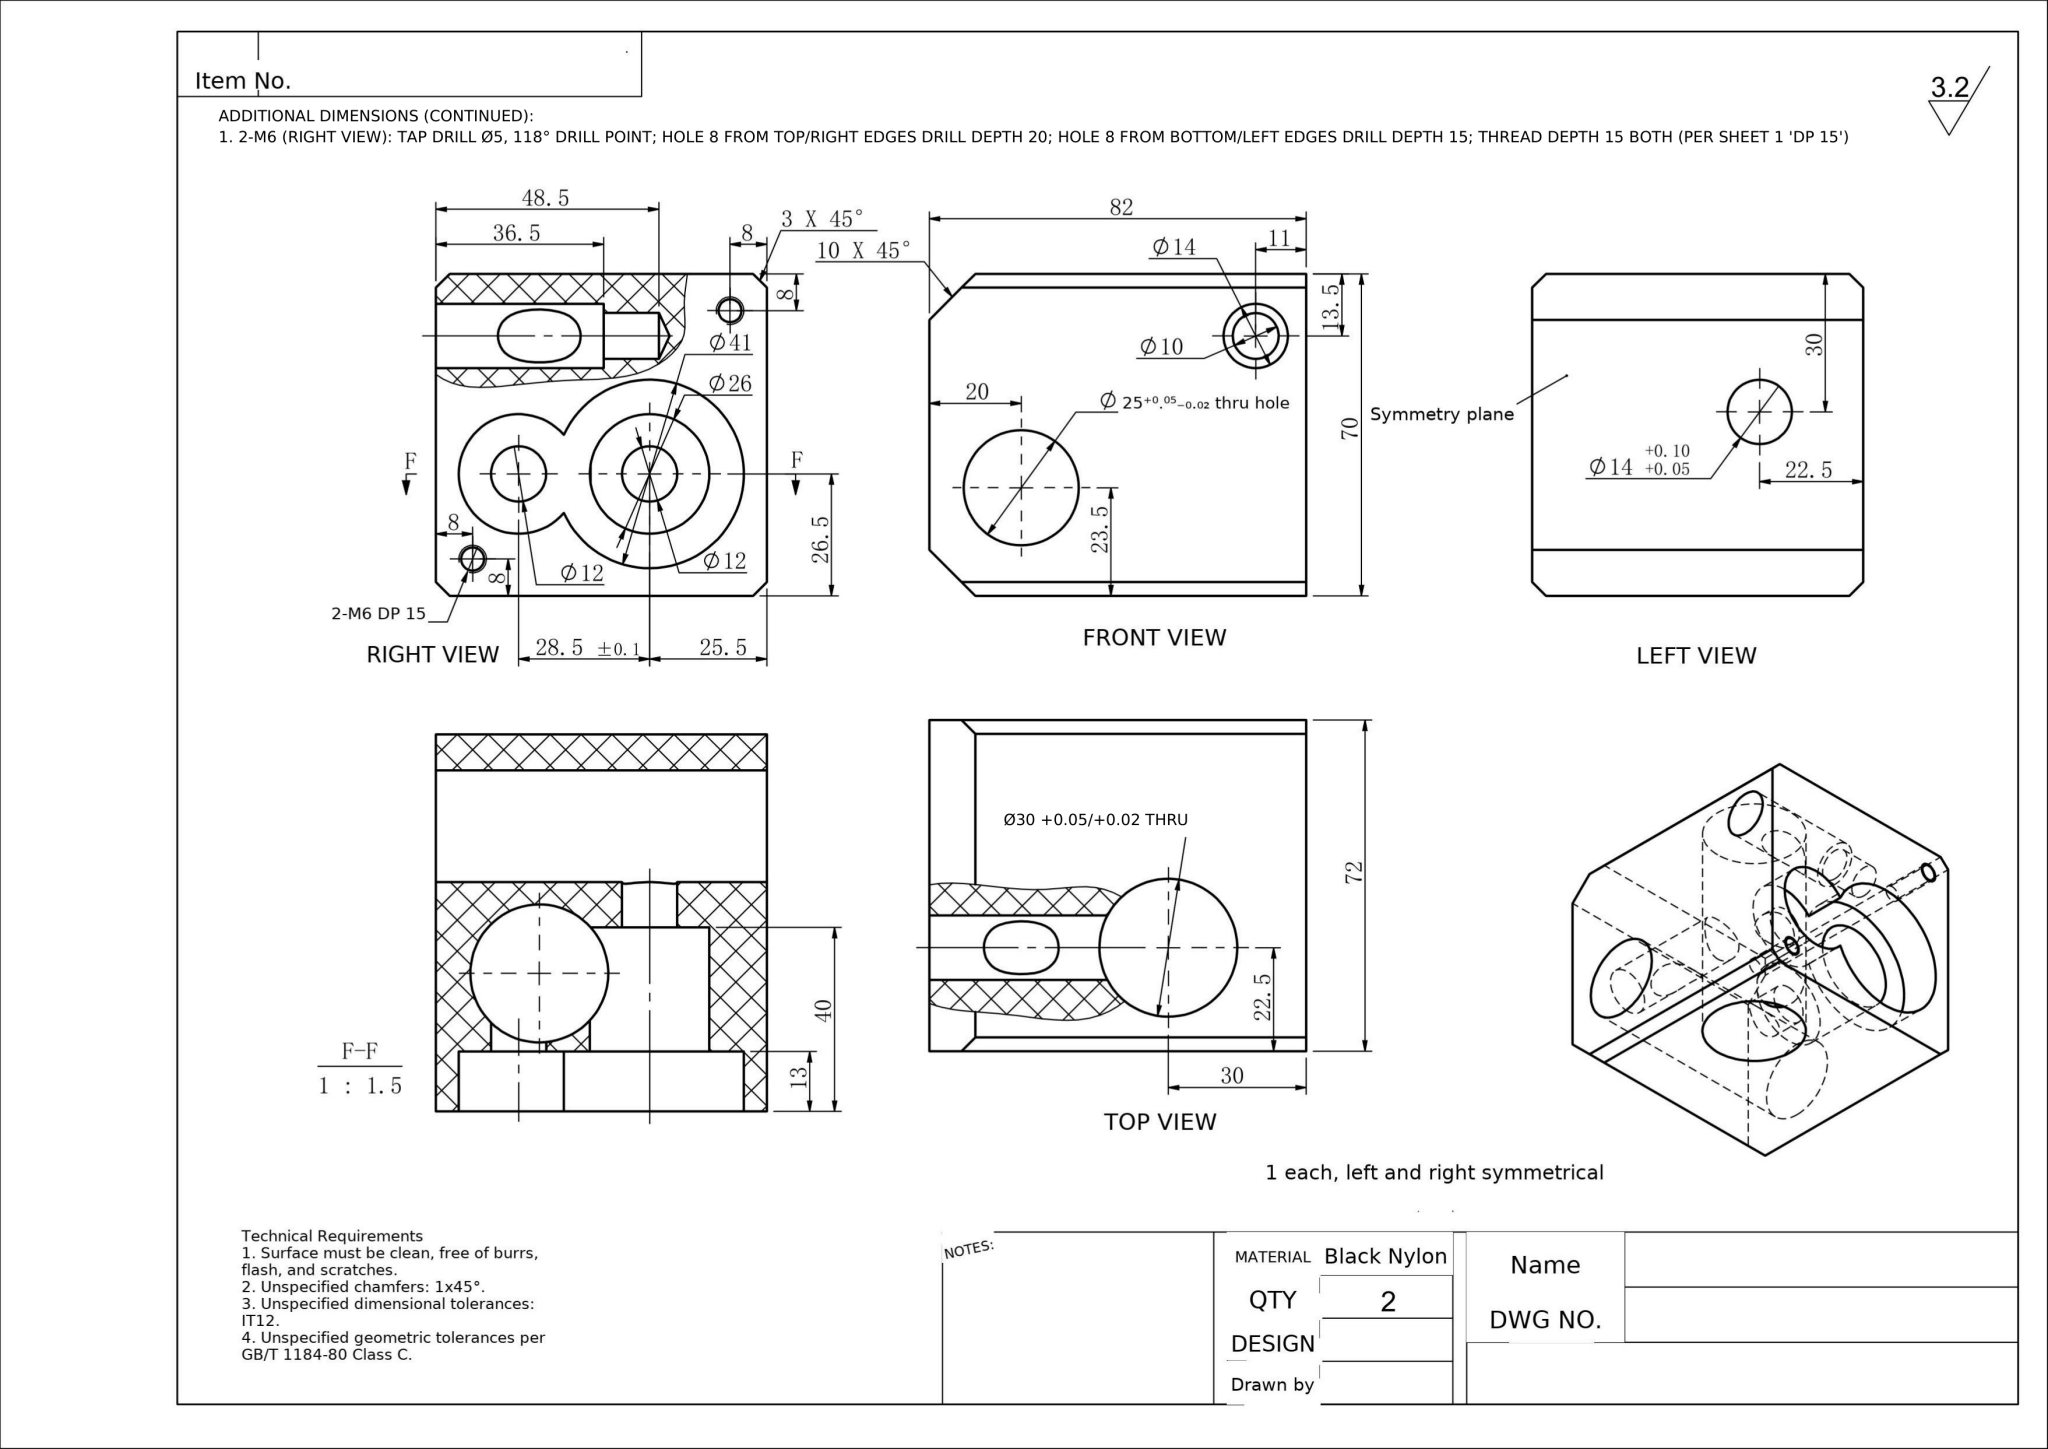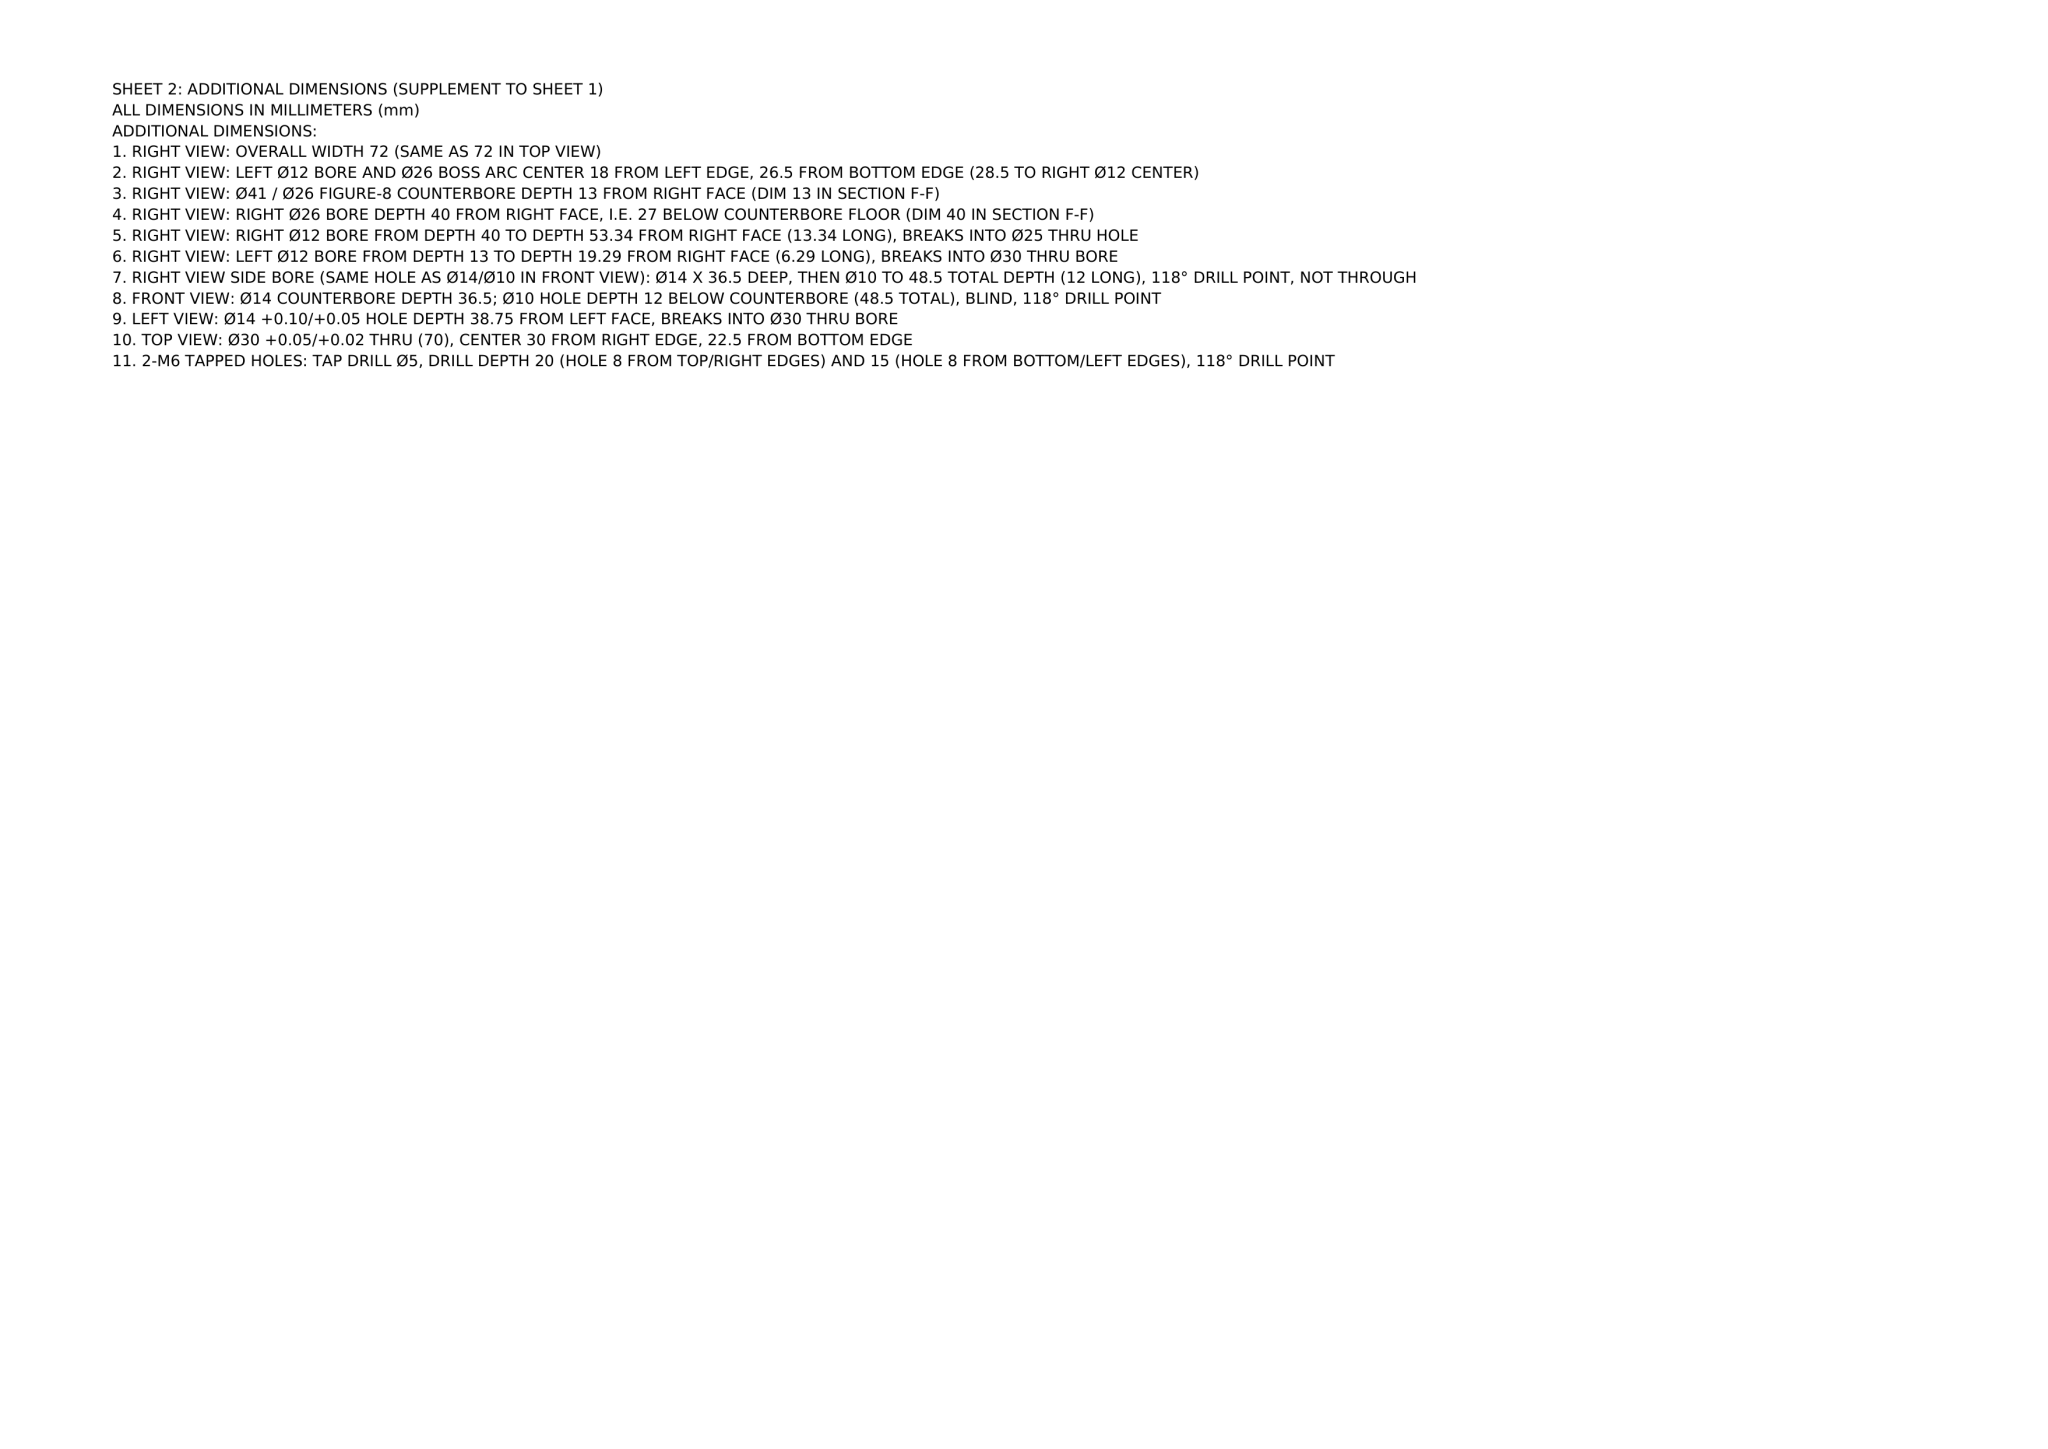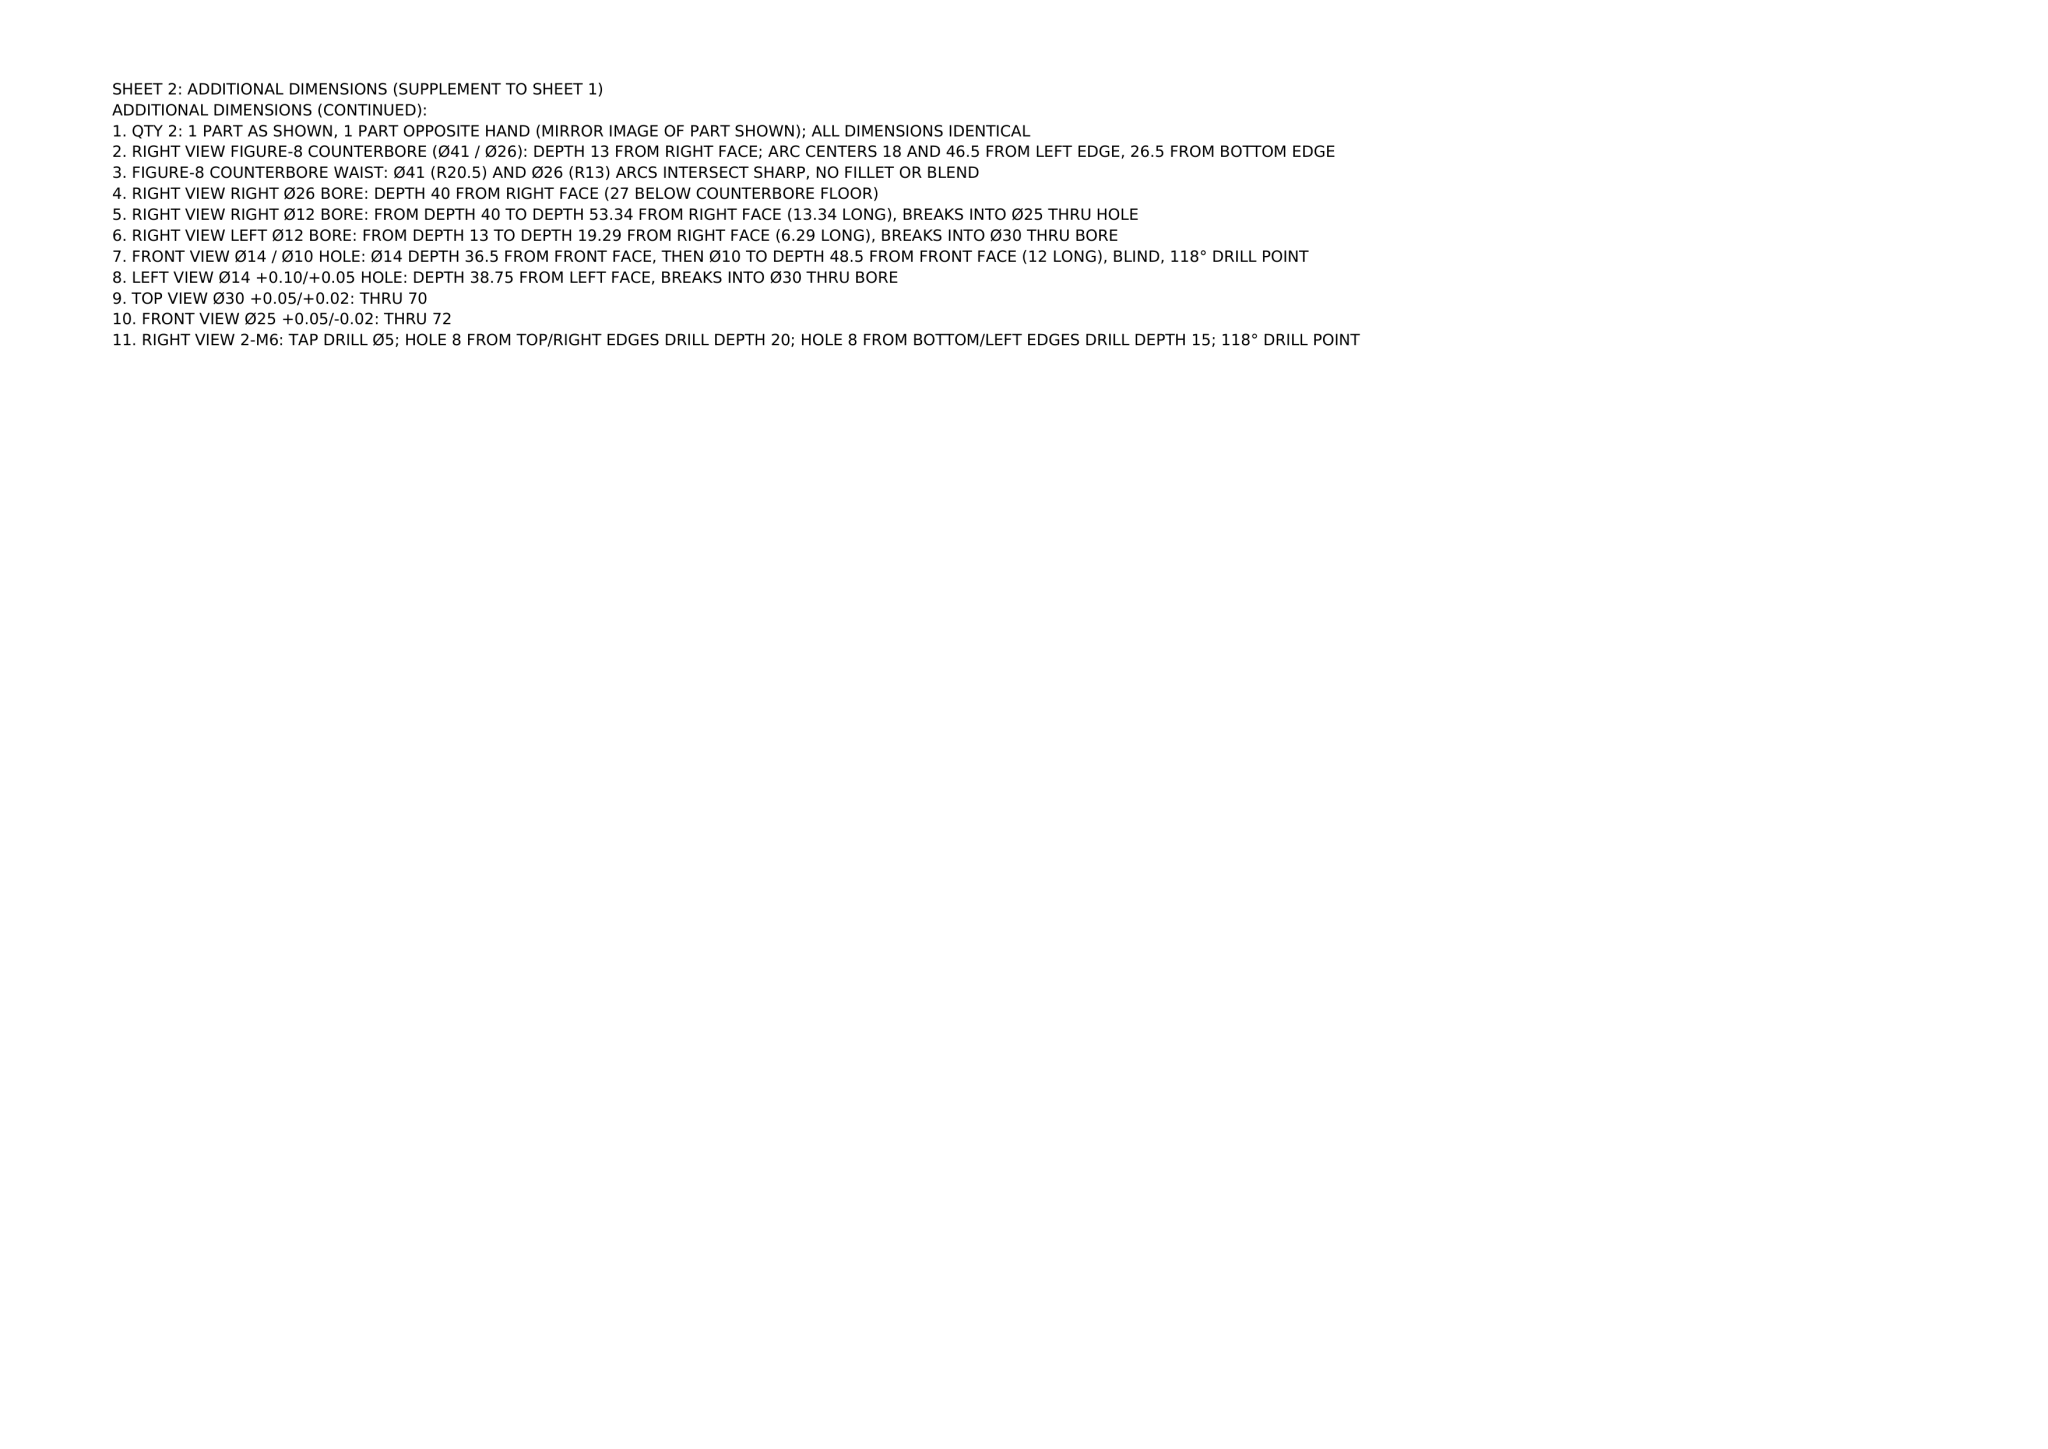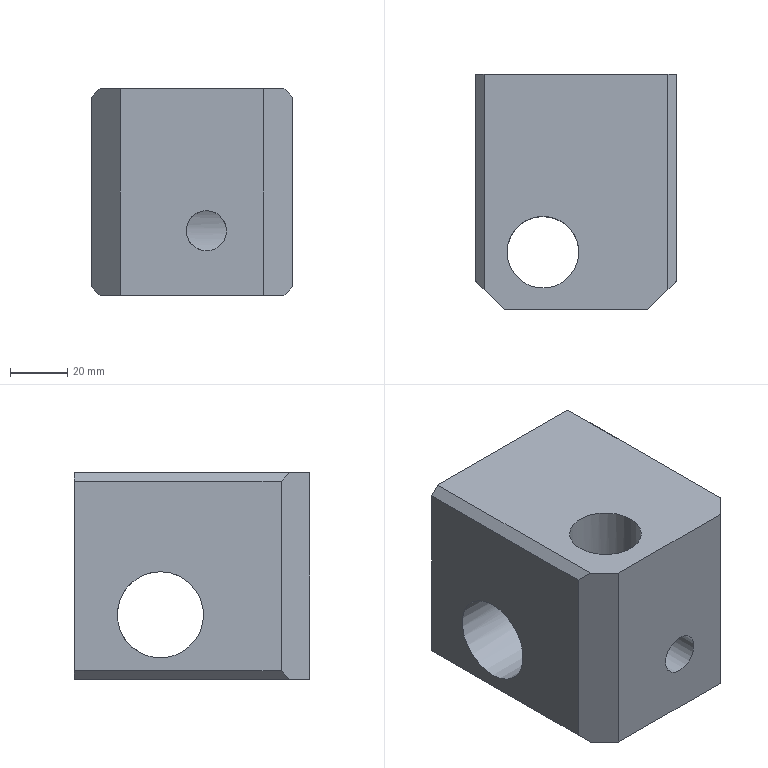Part | NX | mm | 1 solid | 30 faces | box 70 x 82 x 72 mm | volume 268839 mm3 | plane 15 | cylinder 12 | cone 3 | commonest cylinder face diameters 26 x2 5 x2 14 x2 12 x2 41 x1 10 x1 25 x1 30 x1